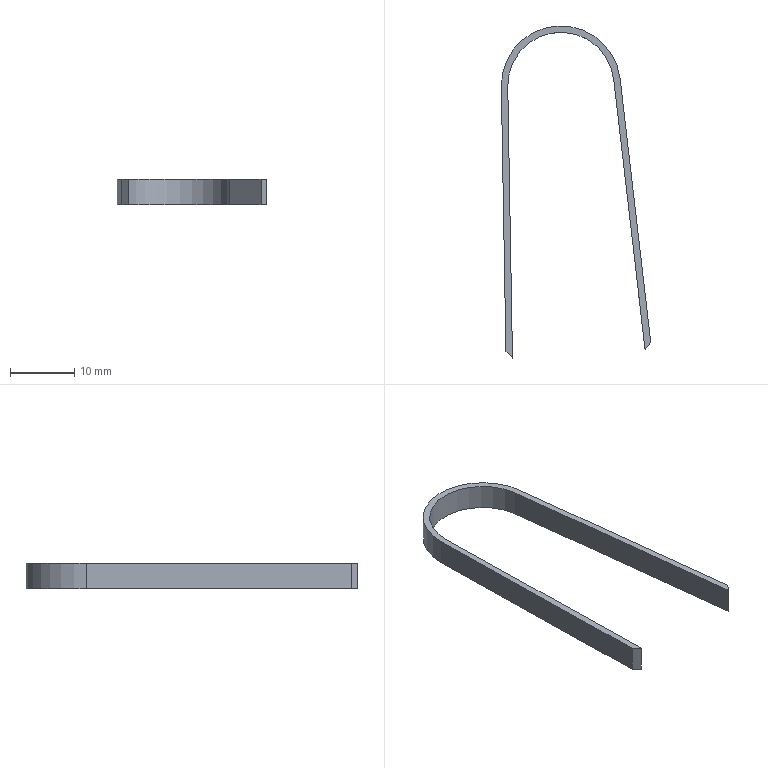Component | SolidWorks | Clip-1 | 1 solid | 10 faces | box 23.23 x 51.65 x 4 mm | volume 441 mm3 | plane 8 | cylinder 2 | commonest cylinder face diameters 16.531 x1 18.531 x1
STEP:
#1=CARTESIAN_POINT('',(-2.639,-1.14,6.23));
#2=VERTEX_POINT('',#1);
#3=CARTESIAN_POINT('',(-2.452,-2.753,6.23));
#4=VERTEX_POINT('',#3);
#5=CARTESIAN_POINT('',(-2.639,-1.14,6.23));
#6=DIRECTION('',(0.1153,-0.9933,-0.));
#7=VECTOR('',#6,39.37);
#8=LINE('',#5,#7);
#9=EDGE_CURVE('',#2,#4,#8,.T.);
#10=ORIENTED_EDGE('',*,*,#9,.T.);
#11=CARTESIAN_POINT('',(-2.452,-2.753,6.073));
#12=VERTEX_POINT('',#11);
#13=CARTESIAN_POINT('',(-2.452,-2.753,6.073));
#14=DIRECTION('',(0.,0.,-1.));
#15=VECTOR('',#14,39.37);
#16=LINE('',#13,#15);
#17=EDGE_CURVE('',#4,#12,#16,.T.);
#18=ORIENTED_EDGE('',*,*,#17,.T.);
#19=CARTESIAN_POINT('',(-2.639,-1.14,6.073));
#20=VERTEX_POINT('',#19);
#21=CARTESIAN_POINT('',(-2.639,-1.14,6.073));
#22=DIRECTION('',(0.1153,-0.9933,-0.));
#23=VECTOR('',#22,39.37);
#24=LINE('',#21,#23);
#25=EDGE_CURVE('',#20,#12,#24,.T.);
#26=ORIENTED_EDGE('',*,*,#25,.F.);
#27=CARTESIAN_POINT('',(-2.639,-1.14,6.073));
#28=DIRECTION('',(-0.,-0.,1.));
#29=VECTOR('',#28,39.37);
#30=LINE('',#27,#29);
#31=EDGE_CURVE('',#20,#2,#30,.T.);
#32=ORIENTED_EDGE('',*,*,#31,.T.);
#33=EDGE_LOOP('',(#10,#18,#26,#32));
#34=FACE_OUTER_BOUND('',#33,.T.);
#35=CARTESIAN_POINT('',(-2.639,-1.14,6.073));
#36=DIRECTION('',(-0.9933,-0.1153,-0.));
#37=DIRECTION('',(-0.1153,0.9933,0.));
#38=AXIS2_PLACEMENT_3D('',#35,#36,#37);
#39=PLANE('',#38);
#40=ADVANCED_FACE('',(#34),#39,.F.);
#41=CARTESIAN_POINT('',(-2.678,-1.144,6.073));
#42=VERTEX_POINT('',#41);
#43=CARTESIAN_POINT('',(-2.487,-2.797,6.073));
#44=VERTEX_POINT('',#43);
#45=CARTESIAN_POINT('',(-2.678,-1.144,6.073));
#46=DIRECTION('',(0.1153,-0.9933,-0.));
#47=VECTOR('',#46,39.37);
#48=LINE('',#45,#47);
#49=EDGE_CURVE('',#42,#44,#48,.T.);
#50=ORIENTED_EDGE('',*,*,#49,.T.);
#51=CARTESIAN_POINT('',(-2.487,-2.797,6.23));
#52=VERTEX_POINT('',#51);
#53=CARTESIAN_POINT('',(-2.487,-2.797,6.073));
#54=DIRECTION('',(-0.,-0.,1.));
#55=VECTOR('',#54,39.37);
#56=LINE('',#53,#55);
#57=EDGE_CURVE('',#44,#52,#56,.T.);
#58=ORIENTED_EDGE('',*,*,#57,.T.);
#59=CARTESIAN_POINT('',(-2.678,-1.144,6.23));
#60=VERTEX_POINT('',#59);
#61=CARTESIAN_POINT('',(-2.678,-1.144,6.23));
#62=DIRECTION('',(0.1153,-0.9933,-0.));
#63=VECTOR('',#62,39.37);
#64=LINE('',#61,#63);
#65=EDGE_CURVE('',#60,#52,#64,.T.);
#66=ORIENTED_EDGE('',*,*,#65,.F.);
#67=CARTESIAN_POINT('',(-2.678,-1.144,6.073));
#68=DIRECTION('',(-0.,-0.,1.));
#69=VECTOR('',#68,39.37);
#70=LINE('',#67,#69);
#71=EDGE_CURVE('',#42,#60,#70,.T.);
#72=ORIENTED_EDGE('',*,*,#71,.F.);
#73=EDGE_LOOP('',(#50,#58,#66,#72));
#74=FACE_OUTER_BOUND('',#73,.T.);
#75=CARTESIAN_POINT('',(-2.678,-1.144,6.073));
#76=DIRECTION('',(-0.9933,-0.1153,-0.));
#77=DIRECTION('',(-0.1153,0.9933,0.));
#78=AXIS2_PLACEMENT_3D('',#75,#76,#77);
#79=PLANE('',#78);
#80=ADVANCED_FACE('',(#74),#79,.T.);
#81=CARTESIAN_POINT('',(-3.327,-1.188,6.23));
#82=VERTEX_POINT('',#81);
#83=CARTESIAN_POINT('',(-3.002,-1.182,6.23));
#84=DIRECTION('',(0.,0.,-1.));
#85=DIRECTION('',(0.9978,0.06638,0.));
#86=AXIS2_PLACEMENT_3D('',#83,#84,#85);
#87=CIRCLE('',#86,0.3254);
#88=EDGE_CURVE('',#82,#60,#87,.T.);
#89=ORIENTED_EDGE('',*,*,#88,.F.);
#90=CARTESIAN_POINT('',(-3.327,-1.188,6.073));
#91=VERTEX_POINT('',#90);
#92=CARTESIAN_POINT('',(-3.327,-1.188,6.073));
#93=DIRECTION('',(-0.,-0.,1.));
#94=VECTOR('',#93,39.37);
#95=LINE('',#92,#94);
#96=EDGE_CURVE('',#91,#82,#95,.T.);
#97=ORIENTED_EDGE('',*,*,#96,.F.);
#98=CARTESIAN_POINT('',(-3.002,-1.182,6.073));
#99=DIRECTION('',(0.,0.,-1.));
#100=DIRECTION('',(0.9978,0.06638,0.));
#101=AXIS2_PLACEMENT_3D('',#98,#99,#100);
#102=CIRCLE('',#101,0.3254);
#103=EDGE_CURVE('',#91,#42,#102,.T.);
#104=ORIENTED_EDGE('',*,*,#103,.T.);
#105=ORIENTED_EDGE('',*,*,#71,.T.);
#106=EDGE_LOOP('',(#89,#97,#104,#105));
#107=FACE_OUTER_BOUND('',#106,.T.);
#108=CARTESIAN_POINT('',(-3.002,-1.182,6.073));
#109=DIRECTION('',(-0.,-0.,1.));
#110=DIRECTION('',(-0.9978,-0.06638,0.));
#111=AXIS2_PLACEMENT_3D('',#108,#109,#110);
#112=CYLINDRICAL_SURFACE('',#111,0.3254);
#113=ADVANCED_FACE('',(#107),#112,.F.);
#114=CARTESIAN_POINT('',(-3.298,-2.851,6.23));
#115=VERTEX_POINT('',#114);
#116=CARTESIAN_POINT('',(-3.327,-1.188,6.23));
#117=DIRECTION('',(-0.01728,0.9999,0.));
#118=VECTOR('',#117,39.37);
#119=LINE('',#116,#118);
#120=EDGE_CURVE('',#115,#82,#119,.T.);
#121=ORIENTED_EDGE('',*,*,#120,.F.);
#122=CARTESIAN_POINT('',(-3.298,-2.851,6.073));
#123=VERTEX_POINT('',#122);
#124=CARTESIAN_POINT('',(-3.298,-2.851,6.073));
#125=DIRECTION('',(0.,0.,-1.));
#126=VECTOR('',#125,39.37);
#127=LINE('',#124,#126);
#128=EDGE_CURVE('',#115,#123,#127,.T.);
#129=ORIENTED_EDGE('',*,*,#128,.T.);
#130=CARTESIAN_POINT('',(-3.327,-1.188,6.073));
#131=DIRECTION('',(-0.01728,0.9999,0.));
#132=VECTOR('',#131,39.37);
#133=LINE('',#130,#132);
#134=EDGE_CURVE('',#123,#91,#133,.T.);
#135=ORIENTED_EDGE('',*,*,#134,.T.);
#136=ORIENTED_EDGE('',*,*,#96,.T.);
#137=EDGE_LOOP('',(#121,#129,#135,#136));
#138=FACE_OUTER_BOUND('',#137,.T.);
#139=CARTESIAN_POINT('',(-3.327,-1.188,6.073));
#140=DIRECTION('',(0.9999,0.01728,0.));
#141=DIRECTION('',(0.01728,-0.9999,-0.));
#142=AXIS2_PLACEMENT_3D('',#139,#140,#141);
#143=PLANE('',#142);
#144=ADVANCED_FACE('',(#138),#143,.T.);
#145=CARTESIAN_POINT('',(-3.338,-2.812,6.073));
#146=VERTEX_POINT('',#145);
#147=CARTESIAN_POINT('',(-3.366,-1.188,6.073));
#148=VERTEX_POINT('',#147);
#149=CARTESIAN_POINT('',(-3.366,-1.188,6.073));
#150=DIRECTION('',(-0.01728,0.9999,0.));
#151=VECTOR('',#150,39.37);
#152=LINE('',#149,#151);
#153=EDGE_CURVE('',#146,#148,#152,.T.);
#154=ORIENTED_EDGE('',*,*,#153,.F.);
#155=CARTESIAN_POINT('',(-3.338,-2.812,6.23));
#156=VERTEX_POINT('',#155);
#157=CARTESIAN_POINT('',(-3.338,-2.812,6.23));
#158=DIRECTION('',(-0.,-0.,1.));
#159=VECTOR('',#158,39.37);
#160=LINE('',#157,#159);
#161=EDGE_CURVE('',#146,#156,#160,.T.);
#162=ORIENTED_EDGE('',*,*,#161,.T.);
#163=CARTESIAN_POINT('',(-3.366,-1.188,6.23));
#164=VERTEX_POINT('',#163);
#165=CARTESIAN_POINT('',(-3.366,-1.188,6.23));
#166=DIRECTION('',(-0.01728,0.9999,0.));
#167=VECTOR('',#166,39.37);
#168=LINE('',#165,#167);
#169=EDGE_CURVE('',#156,#164,#168,.T.);
#170=ORIENTED_EDGE('',*,*,#169,.T.);
#171=CARTESIAN_POINT('',(-3.366,-1.188,6.073));
#172=DIRECTION('',(-0.,-0.,1.));
#173=VECTOR('',#172,39.37);
#174=LINE('',#171,#173);
#175=EDGE_CURVE('',#148,#164,#174,.T.);
#176=ORIENTED_EDGE('',*,*,#175,.F.);
#177=EDGE_LOOP('',(#154,#162,#170,#176));
#178=FACE_OUTER_BOUND('',#177,.T.);
#179=CARTESIAN_POINT('',(-3.366,-1.188,6.073));
#180=DIRECTION('',(0.9999,0.01728,0.));
#181=DIRECTION('',(0.01728,-0.9999,-0.));
#182=AXIS2_PLACEMENT_3D('',#179,#180,#181);
#183=PLANE('',#182);
#184=ADVANCED_FACE('',(#178),#183,.F.);
#185=CARTESIAN_POINT('',(-3.002,-1.182,6.23));
#186=DIRECTION('',(0.,0.,-1.));
#187=DIRECTION('',(0.9978,0.06638,0.));
#188=AXIS2_PLACEMENT_3D('',#185,#186,#187);
#189=CIRCLE('',#188,0.3648);
#190=EDGE_CURVE('',#164,#2,#189,.T.);
#191=ORIENTED_EDGE('',*,*,#190,.T.);
#192=ORIENTED_EDGE('',*,*,#31,.F.);
#193=CARTESIAN_POINT('',(-3.002,-1.182,6.073));
#194=DIRECTION('',(0.,0.,-1.));
#195=DIRECTION('',(0.9978,0.06638,0.));
#196=AXIS2_PLACEMENT_3D('',#193,#194,#195);
#197=CIRCLE('',#196,0.3648);
#198=EDGE_CURVE('',#148,#20,#197,.T.);
#199=ORIENTED_EDGE('',*,*,#198,.F.);
#200=ORIENTED_EDGE('',*,*,#175,.T.);
#201=EDGE_LOOP('',(#191,#192,#199,#200));
#202=FACE_OUTER_BOUND('',#201,.T.);
#203=CARTESIAN_POINT('',(-3.002,-1.182,6.073));
#204=DIRECTION('',(-0.,-0.,1.));
#205=DIRECTION('',(-0.9978,-0.06638,0.));
#206=AXIS2_PLACEMENT_3D('',#203,#204,#205);
#207=CYLINDRICAL_SURFACE('',#206,0.3648);
#208=ADVANCED_FACE('',(#202),#207,.T.);
#209=ORIENTED_EDGE('',*,*,#25,.T.);
#210=CARTESIAN_POINT('',(-1.899,-2.055,6.073));
#211=DIRECTION('',(-0.6208,-0.7839,-0.));
#212=VECTOR('',#211,39.37);
#213=LINE('',#210,#212);
#214=EDGE_CURVE('',#12,#44,#213,.T.);
#215=ORIENTED_EDGE('',*,*,#214,.T.);
#216=ORIENTED_EDGE('',*,*,#49,.F.);
#217=ORIENTED_EDGE('',*,*,#103,.F.);
#218=ORIENTED_EDGE('',*,*,#134,.F.);
#219=CARTESIAN_POINT('',(-3.979,-2.193,6.073));
#220=DIRECTION('',(-0.7192,0.6948,0.));
#221=VECTOR('',#220,39.37);
#222=LINE('',#219,#221);
#223=EDGE_CURVE('',#123,#146,#222,.T.);
#224=ORIENTED_EDGE('',*,*,#223,.T.);
#225=ORIENTED_EDGE('',*,*,#153,.T.);
#226=ORIENTED_EDGE('',*,*,#198,.T.);
#227=EDGE_LOOP('',(#209,#215,#216,#217,#218,#224,#225,#226));
#228=FACE_OUTER_BOUND('',#227,.T.);
#229=CARTESIAN_POINT('',(-3.002,-1.182,6.073));
#230=DIRECTION('',(0.,0.,-1.));
#231=DIRECTION('',(0.9978,0.06638,0.));
#232=AXIS2_PLACEMENT_3D('',#229,#230,#231);
#233=PLANE('',#232);
#234=ADVANCED_FACE('',(#228),#233,.T.);
#235=ORIENTED_EDGE('',*,*,#65,.T.);
#236=CARTESIAN_POINT('',(-2.556,-2.884,6.23));
#237=DIRECTION('',(0.6208,0.7839,0.));
#238=VECTOR('',#237,39.37);
#239=LINE('',#236,#238);
#240=EDGE_CURVE('',#52,#4,#239,.T.);
#241=ORIENTED_EDGE('',*,*,#240,.T.);
#242=ORIENTED_EDGE('',*,*,#9,.F.);
#243=ORIENTED_EDGE('',*,*,#190,.F.);
#244=ORIENTED_EDGE('',*,*,#169,.F.);
#245=CARTESIAN_POINT('',(-3.338,-2.812,6.23));
#246=DIRECTION('',(0.7192,-0.6948,-0.));
#247=VECTOR('',#246,39.37);
#248=LINE('',#245,#247);
#249=EDGE_CURVE('',#156,#115,#248,.T.);
#250=ORIENTED_EDGE('',*,*,#249,.T.);
#251=ORIENTED_EDGE('',*,*,#120,.T.);
#252=ORIENTED_EDGE('',*,*,#88,.T.);
#253=EDGE_LOOP('',(#235,#241,#242,#243,#244,#250,#251,#252));
#254=FACE_OUTER_BOUND('',#253,.T.);
#255=CARTESIAN_POINT('',(-3.002,-1.182,6.23));
#256=DIRECTION('',(0.,0.,-1.));
#257=DIRECTION('',(0.9978,0.06638,0.));
#258=AXIS2_PLACEMENT_3D('',#255,#256,#257);
#259=PLANE('',#258);
#260=ADVANCED_FACE('',(#254),#259,.F.);
#261=ORIENTED_EDGE('',*,*,#223,.F.);
#262=ORIENTED_EDGE('',*,*,#128,.F.);
#263=ORIENTED_EDGE('',*,*,#249,.F.);
#264=ORIENTED_EDGE('',*,*,#161,.F.);
#265=EDGE_LOOP('',(#261,#262,#263,#264));
#266=FACE_OUTER_BOUND('',#265,.T.);
#267=CARTESIAN_POINT('',(-3.338,-2.812,6.073));
#268=DIRECTION('',(-0.6948,-0.7192,-0.));
#269=DIRECTION('',(0.,0.,-1.));
#270=AXIS2_PLACEMENT_3D('',#267,#268,#269);
#271=PLANE('',#270);
#272=ADVANCED_FACE('',(#266),#271,.T.);
#273=ORIENTED_EDGE('',*,*,#214,.F.);
#274=ORIENTED_EDGE('',*,*,#17,.F.);
#275=ORIENTED_EDGE('',*,*,#240,.F.);
#276=ORIENTED_EDGE('',*,*,#57,.F.);
#277=EDGE_LOOP('',(#273,#274,#275,#276));
#278=FACE_OUTER_BOUND('',#277,.T.);
#279=CARTESIAN_POINT('',(-2.556,-2.884,6.073));
#280=DIRECTION('',(0.7839,-0.6208,-0.));
#281=DIRECTION('',(0.,0.,-1.));
#282=AXIS2_PLACEMENT_3D('',#279,#280,#281);
#283=PLANE('',#282);
#284=ADVANCED_FACE('',(#278),#283,.T.);
#285=CLOSED_SHELL('',(#40,#80,#113,#144,#184,#208,#234,#260,#272,#284));
#286=MANIFOLD_SOLID_BREP('',#285);
#287=CARTESIAN_POINT('',(0.,0.,0.));
#288=DIRECTION('',(0.,0.,1.));
#289=DIRECTION('',(1.,0.,0.));
#290=AXIS2_PLACEMENT_3D('',#287,#288,#289);
#291=(LENGTH_UNIT()NAMED_UNIT(*)SI_UNIT($,.METRE.));
#292=LENGTH_MEASURE_WITH_UNIT(LENGTH_MEASURE(0.0254),#291);
#293=DIMENSIONAL_EXPONENTS(1.,0.,0.,0.,0.,0.,0.);
#294=(CONVERSION_BASED_UNIT('',#292)LENGTH_UNIT()NAMED_UNIT(#293));
#295=UNCERTAINTY_MEASURE_WITH_UNIT(LENGTH_MEASURE(0.00001),#294,'','');
#296=(NAMED_UNIT(*)PLANE_ANGLE_UNIT()SI_UNIT($,.RADIAN.));
#297=(NAMED_UNIT(*)SI_UNIT($,.STERADIAN.)SOLID_ANGLE_UNIT());
#298=(GEOMETRIC_REPRESENTATION_CONTEXT(3)GLOBAL_UNCERTAINTY_ASSIGNED_CONTEXT((#295))GLOBAL_UNIT_ASSIGNED_CONTEXT((#294,#296,#297))REPRESENTATION_CONTEXT('',''));
#299=ADVANCED_BREP_SHAPE_REPRESENTATION('',(#286,#290),#298);
#300=COLOUR_RGB('',0.7922,0.8196,0.9333);
#301=FILL_AREA_STYLE_COLOUR('',#300);
#302=FILL_AREA_STYLE('',(#301));
#303=SURFACE_STYLE_FILL_AREA(#302);
#304=SURFACE_SIDE_STYLE('',(#303));
#305=SURFACE_STYLE_USAGE(.BOTH.,#304);
#306=PRESENTATION_STYLE_ASSIGNMENT((#305));
#307=STYLED_ITEM('',(#306),#286);
#308=(LENGTH_UNIT()NAMED_UNIT(*)SI_UNIT($,.METRE.));
#309=LENGTH_MEASURE_WITH_UNIT(LENGTH_MEASURE(0.0254),#308);
#310=DIMENSIONAL_EXPONENTS(1.,0.,0.,0.,0.,0.,0.);
#311=(CONVERSION_BASED_UNIT('',#309)LENGTH_UNIT()NAMED_UNIT(#310));
#312=UNCERTAINTY_MEASURE_WITH_UNIT(LENGTH_MEASURE(0.00001),#311,'','');
#313=(NAMED_UNIT(*)PLANE_ANGLE_UNIT()SI_UNIT($,.RADIAN.));
#314=(NAMED_UNIT(*)SI_UNIT($,.STERADIAN.)SOLID_ANGLE_UNIT());
#315=(GEOMETRIC_REPRESENTATION_CONTEXT(3)GLOBAL_UNCERTAINTY_ASSIGNED_CONTEXT((#312))GLOBAL_UNIT_ASSIGNED_CONTEXT((#311,#313,#314))REPRESENTATION_CONTEXT('',''));
#316=MECHANICAL_DESIGN_GEOMETRIC_PRESENTATION_REPRESENTATION('',(#307),#315);
#317=PRESENTATION_LAYER_ASSIGNMENT('','',(#307));